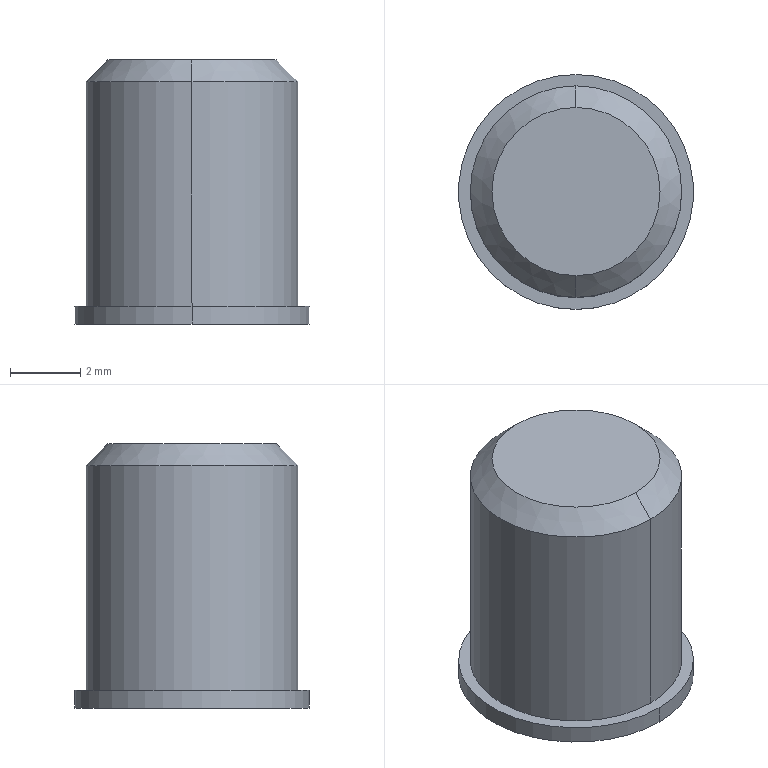Component | SolidWorks | NewCurveBenderHG20Slider-DoubleWheel-1_NewTypeCurveBenderDoubleWheel-1 | 1 solid | 16 faces | box 6.67 x 6.67 x 7.5 mm | volume 204 mm3 | plane 10 | cylinder 4 | cone 2 | commonest cylinder face diameters 6 x2 6.667 x2
STEP:
#1=COLOUR_RGB('',0.7922,0.8196,0.9333);
#2=FILL_AREA_STYLE_COLOUR('',#1);
#3=FILL_AREA_STYLE('',(#2));
#4=SURFACE_STYLE_FILL_AREA(#3);
#5=SURFACE_SIDE_STYLE('',(#4));
#6=SURFACE_STYLE_USAGE(.BOTH.,#5);
#7=PRESENTATION_STYLE_ASSIGNMENT((#6));
#8=CARTESIAN_POINT('',(3.15,1.417,2.082));
#9=VERTEX_POINT('',#8);
#10=CARTESIAN_POINT('',(3.15,1.654,2.082));
#11=VERTEX_POINT('',#10);
#12=CARTESIAN_POINT('',(3.15,1.535,2.082));
#13=DIRECTION('',(-0.,0.,1.));
#14=DIRECTION('',(0.,-1.,0.));
#15=AXIS2_PLACEMENT_3D('',#12,#13,#14);
#16=CIRCLE('',#15,0.1181);
#17=EDGE_CURVE('',#9,#11,#16,.T.);
#18=ORIENTED_EDGE('',*,*,#17,.T.);
#19=CARTESIAN_POINT('',(3.15,1.654,2.333));
#20=VERTEX_POINT('',#19);
#21=CARTESIAN_POINT('',(3.15,1.654,2.062));
#22=DIRECTION('',(-0.,0.,1.));
#23=VECTOR('',#22,39.37);
#24=LINE('',#21,#23);
#25=EDGE_CURVE('',#11,#20,#24,.T.);
#26=ORIENTED_EDGE('',*,*,#25,.T.);
#27=CARTESIAN_POINT('',(3.15,1.417,2.333));
#28=VERTEX_POINT('',#27);
#29=CARTESIAN_POINT('',(3.15,1.535,2.333));
#30=DIRECTION('',(0.,0.,-1.));
#31=DIRECTION('',(0.,-1.,0.));
#32=AXIS2_PLACEMENT_3D('',#29,#30,#31);
#33=CIRCLE('',#32,0.1181);
#34=EDGE_CURVE('',#20,#28,#33,.T.);
#35=ORIENTED_EDGE('',*,*,#34,.T.);
#36=CARTESIAN_POINT('',(3.15,1.417,2.062));
#37=DIRECTION('',(-0.,0.,1.));
#38=VECTOR('',#37,39.37);
#39=LINE('',#36,#38);
#40=EDGE_CURVE('',#9,#28,#39,.T.);
#41=ORIENTED_EDGE('',*,*,#40,.F.);
#42=EDGE_LOOP('',(#18,#26,#35,#41));
#43=FACE_OUTER_BOUND('',#42,.T.);
#44=CARTESIAN_POINT('',(3.15,1.535,2.062));
#45=DIRECTION('',(-0.,0.,1.));
#46=DIRECTION('',(0.,-1.,0.));
#47=AXIS2_PLACEMENT_3D('',#44,#45,#46);
#48=CYLINDRICAL_SURFACE('',#47,0.1181);
#49=ADVANCED_FACE('',(#43),#48,.T.);
#50=CARTESIAN_POINT('',(3.15,1.629,2.357));
#51=VERTEX_POINT('',#50);
#52=CARTESIAN_POINT('',(3.15,1.441,2.357));
#53=VERTEX_POINT('',#52);
#54=CARTESIAN_POINT('',(3.15,1.535,2.357));
#55=DIRECTION('',(0.,0.,-1.));
#56=DIRECTION('',(0.,1.,0.));
#57=AXIS2_PLACEMENT_3D('',#54,#55,#56);
#58=CIRCLE('',#57,0.09396);
#59=EDGE_CURVE('',#51,#53,#58,.T.);
#60=ORIENTED_EDGE('',*,*,#59,.T.);
#61=CARTESIAN_POINT('',(3.15,1.417,2.333));
#62=DIRECTION('',(0.,-0.7071,-0.7071));
#63=VECTOR('',#62,39.37);
#64=LINE('',#61,#63);
#65=EDGE_CURVE('',#53,#28,#64,.T.);
#66=ORIENTED_EDGE('',*,*,#65,.T.);
#67=ORIENTED_EDGE('',*,*,#34,.F.);
#68=CARTESIAN_POINT('',(3.15,1.654,2.333));
#69=DIRECTION('',(0.,0.7071,-0.7071));
#70=VECTOR('',#69,39.37);
#71=LINE('',#68,#70);
#72=EDGE_CURVE('',#51,#20,#71,.T.);
#73=ORIENTED_EDGE('',*,*,#72,.F.);
#74=EDGE_LOOP('',(#60,#66,#67,#73));
#75=FACE_OUTER_BOUND('',#74,.T.);
#76=CARTESIAN_POINT('',(3.15,1.535,2.333));
#77=DIRECTION('',(0.,0.,-1.));
#78=DIRECTION('',(0.,1.,0.));
#79=AXIS2_PLACEMENT_3D('',#76,#77,#78);
#80=CONICAL_SURFACE('',#79,0.1181,0.7854);
#81=ADVANCED_FACE('',(#75),#80,.T.);
#82=CARTESIAN_POINT('',(3.15,1.404,2.062));
#83=VERTEX_POINT('',#82);
#84=CARTESIAN_POINT('',(3.15,1.667,2.062));
#85=VERTEX_POINT('',#84);
#86=CARTESIAN_POINT('',(3.15,1.535,2.062));
#87=DIRECTION('',(-0.,0.,1.));
#88=DIRECTION('',(0.,-1.,0.));
#89=AXIS2_PLACEMENT_3D('',#86,#87,#88);
#90=CIRCLE('',#89,0.1312);
#91=EDGE_CURVE('',#83,#85,#90,.T.);
#92=ORIENTED_EDGE('',*,*,#91,.T.);
#93=CARTESIAN_POINT('',(3.15,1.667,2.082));
#94=VERTEX_POINT('',#93);
#95=CARTESIAN_POINT('',(3.15,1.667,2.062));
#96=DIRECTION('',(-0.,0.,1.));
#97=VECTOR('',#96,39.37);
#98=LINE('',#95,#97);
#99=EDGE_CURVE('',#85,#94,#98,.T.);
#100=ORIENTED_EDGE('',*,*,#99,.T.);
#101=CARTESIAN_POINT('',(3.15,1.404,2.082));
#102=VERTEX_POINT('',#101);
#103=CARTESIAN_POINT('',(3.15,1.535,2.082));
#104=DIRECTION('',(0.,0.,-1.));
#105=DIRECTION('',(0.,-1.,0.));
#106=AXIS2_PLACEMENT_3D('',#103,#104,#105);
#107=CIRCLE('',#106,0.1312);
#108=EDGE_CURVE('',#94,#102,#107,.T.);
#109=ORIENTED_EDGE('',*,*,#108,.T.);
#110=CARTESIAN_POINT('',(3.15,1.404,2.062));
#111=DIRECTION('',(-0.,0.,1.));
#112=VECTOR('',#111,39.37);
#113=LINE('',#110,#112);
#114=EDGE_CURVE('',#83,#102,#113,.T.);
#115=ORIENTED_EDGE('',*,*,#114,.F.);
#116=EDGE_LOOP('',(#92,#100,#109,#115));
#117=FACE_OUTER_BOUND('',#116,.T.);
#118=CARTESIAN_POINT('',(3.15,1.535,2.062));
#119=DIRECTION('',(-0.,0.,1.));
#120=DIRECTION('',(0.,-1.,0.));
#121=AXIS2_PLACEMENT_3D('',#118,#119,#120);
#122=CYLINDRICAL_SURFACE('',#121,0.1312);
#123=ADVANCED_FACE('',(#117),#122,.T.);
#124=ORIENTED_EDGE('',*,*,#25,.F.);
#125=CARTESIAN_POINT('',(3.15,1.535,2.082));
#126=DIRECTION('',(-0.,0.,1.));
#127=DIRECTION('',(0.,-1.,0.));
#128=AXIS2_PLACEMENT_3D('',#125,#126,#127);
#129=CIRCLE('',#128,0.1181);
#130=EDGE_CURVE('',#11,#9,#129,.T.);
#131=ORIENTED_EDGE('',*,*,#130,.T.);
#132=ORIENTED_EDGE('',*,*,#40,.T.);
#133=CARTESIAN_POINT('',(3.15,1.535,2.333));
#134=DIRECTION('',(0.,0.,-1.));
#135=DIRECTION('',(0.,-1.,0.));
#136=AXIS2_PLACEMENT_3D('',#133,#134,#135);
#137=CIRCLE('',#136,0.1181);
#138=EDGE_CURVE('',#28,#20,#137,.T.);
#139=ORIENTED_EDGE('',*,*,#138,.T.);
#140=EDGE_LOOP('',(#124,#131,#132,#139));
#141=FACE_OUTER_BOUND('',#140,.T.);
#142=CARTESIAN_POINT('',(3.15,1.535,2.062));
#143=DIRECTION('',(-0.,0.,1.));
#144=DIRECTION('',(0.,-1.,0.));
#145=AXIS2_PLACEMENT_3D('',#142,#143,#144);
#146=CYLINDRICAL_SURFACE('',#145,0.1181);
#147=ADVANCED_FACE('',(#141),#146,.T.);
#148=ORIENTED_EDGE('',*,*,#65,.F.);
#149=CARTESIAN_POINT('',(3.15,1.535,2.357));
#150=DIRECTION('',(0.,0.,-1.));
#151=DIRECTION('',(0.,1.,0.));
#152=AXIS2_PLACEMENT_3D('',#149,#150,#151);
#153=CIRCLE('',#152,0.09396);
#154=EDGE_CURVE('',#53,#51,#153,.T.);
#155=ORIENTED_EDGE('',*,*,#154,.T.);
#156=ORIENTED_EDGE('',*,*,#72,.T.);
#157=ORIENTED_EDGE('',*,*,#138,.F.);
#158=EDGE_LOOP('',(#148,#155,#156,#157));
#159=FACE_OUTER_BOUND('',#158,.T.);
#160=CARTESIAN_POINT('',(3.15,1.535,2.333));
#161=DIRECTION('',(0.,0.,-1.));
#162=DIRECTION('',(0.,1.,0.));
#163=AXIS2_PLACEMENT_3D('',#160,#161,#162);
#164=CONICAL_SURFACE('',#163,0.1181,0.7854);
#165=ADVANCED_FACE('',(#159),#164,.T.);
#166=ORIENTED_EDGE('',*,*,#17,.F.);
#167=ORIENTED_EDGE('',*,*,#130,.F.);
#168=EDGE_LOOP('',(#166,#167));
#169=FACE_BOUND('',#168,.T.);
#170=CARTESIAN_POINT('',(3.15,1.535,2.082));
#171=DIRECTION('',(0.,0.,-1.));
#172=DIRECTION('',(0.,-1.,0.));
#173=AXIS2_PLACEMENT_3D('',#170,#171,#172);
#174=CIRCLE('',#173,0.1312);
#175=EDGE_CURVE('',#102,#94,#174,.T.);
#176=ORIENTED_EDGE('',*,*,#175,.F.);
#177=ORIENTED_EDGE('',*,*,#108,.F.);
#178=EDGE_LOOP('',(#176,#177));
#179=FACE_OUTER_BOUND('',#178,.T.);
#180=CARTESIAN_POINT('',(3.031,1.535,2.082));
#181=DIRECTION('',(0.,0.,-1.));
#182=DIRECTION('',(0.,1.,0.));
#183=AXIS2_PLACEMENT_3D('',#180,#181,#182);
#184=PLANE('',#183);
#185=ADVANCED_FACE('',(#169,#179),#184,.F.);
#186=ORIENTED_EDGE('',*,*,#59,.F.);
#187=ORIENTED_EDGE('',*,*,#154,.F.);
#188=EDGE_LOOP('',(#186,#187));
#189=FACE_OUTER_BOUND('',#188,.T.);
#190=CARTESIAN_POINT('',(3.15,1.535,2.357));
#191=DIRECTION('',(0.,0.,-1.));
#192=DIRECTION('',(0.,1.,0.));
#193=AXIS2_PLACEMENT_3D('',#190,#191,#192);
#194=PLANE('',#193);
#195=ADVANCED_FACE('',(#189),#194,.F.);
#196=ORIENTED_EDGE('',*,*,#99,.F.);
#197=CARTESIAN_POINT('',(3.15,1.535,2.062));
#198=DIRECTION('',(-0.,0.,1.));
#199=DIRECTION('',(0.,-1.,0.));
#200=AXIS2_PLACEMENT_3D('',#197,#198,#199);
#201=CIRCLE('',#200,0.1312);
#202=EDGE_CURVE('',#85,#83,#201,.T.);
#203=ORIENTED_EDGE('',*,*,#202,.T.);
#204=ORIENTED_EDGE('',*,*,#114,.T.);
#205=ORIENTED_EDGE('',*,*,#175,.T.);
#206=EDGE_LOOP('',(#196,#203,#204,#205));
#207=FACE_OUTER_BOUND('',#206,.T.);
#208=CARTESIAN_POINT('',(3.15,1.535,2.062));
#209=DIRECTION('',(-0.,0.,1.));
#210=DIRECTION('',(0.,-1.,0.));
#211=AXIS2_PLACEMENT_3D('',#208,#209,#210);
#212=CYLINDRICAL_SURFACE('',#211,0.1312);
#213=ADVANCED_FACE('',(#207),#212,.T.);
#214=ORIENTED_EDGE('',*,*,#91,.F.);
#215=ORIENTED_EDGE('',*,*,#202,.F.);
#216=EDGE_LOOP('',(#214,#215));
#217=FACE_OUTER_BOUND('',#216,.T.);
#218=CARTESIAN_POINT('',(3.15,1.454,2.062));
#219=VERTEX_POINT('',#218);
#220=CARTESIAN_POINT('',(3.079,1.495,2.062));
#221=VERTEX_POINT('',#220);
#222=CARTESIAN_POINT('',(3.15,1.454,2.062));
#223=DIRECTION('',(-0.866,0.5,-0.));
#224=VECTOR('',#223,39.37);
#225=LINE('',#222,#224);
#226=EDGE_CURVE('',#219,#221,#225,.T.);
#227=ORIENTED_EDGE('',*,*,#226,.F.);
#228=CARTESIAN_POINT('',(3.22,1.495,2.062));
#229=VERTEX_POINT('',#228);
#230=CARTESIAN_POINT('',(3.22,1.495,2.062));
#231=DIRECTION('',(-0.866,-0.5,-0.));
#232=VECTOR('',#231,39.37);
#233=LINE('',#230,#232);
#234=EDGE_CURVE('',#229,#219,#233,.T.);
#235=ORIENTED_EDGE('',*,*,#234,.F.);
#236=CARTESIAN_POINT('',(3.22,1.576,2.062));
#237=VERTEX_POINT('',#236);
#238=CARTESIAN_POINT('',(3.22,1.535,2.062));
#239=DIRECTION('',(0.,-1.,0.));
#240=VECTOR('',#239,39.37);
#241=LINE('',#238,#240);
#242=EDGE_CURVE('',#237,#229,#241,.T.);
#243=ORIENTED_EDGE('',*,*,#242,.F.);
#244=CARTESIAN_POINT('',(3.15,1.617,2.062));
#245=VERTEX_POINT('',#244);
#246=CARTESIAN_POINT('',(3.15,1.617,2.062));
#247=DIRECTION('',(0.866,-0.5,0.));
#248=VECTOR('',#247,39.37);
#249=LINE('',#246,#248);
#250=EDGE_CURVE('',#245,#237,#249,.T.);
#251=ORIENTED_EDGE('',*,*,#250,.F.);
#252=CARTESIAN_POINT('',(3.079,1.576,2.062));
#253=VERTEX_POINT('',#252);
#254=CARTESIAN_POINT('',(3.079,1.576,2.062));
#255=DIRECTION('',(0.866,0.5,0.));
#256=VECTOR('',#255,39.37);
#257=LINE('',#254,#256);
#258=EDGE_CURVE('',#253,#245,#257,.T.);
#259=ORIENTED_EDGE('',*,*,#258,.F.);
#260=CARTESIAN_POINT('',(3.079,1.535,2.062));
#261=DIRECTION('',(0.,1.,0.));
#262=VECTOR('',#261,39.37);
#263=LINE('',#260,#262);
#264=EDGE_CURVE('',#221,#253,#263,.T.);
#265=ORIENTED_EDGE('',*,*,#264,.F.);
#266=EDGE_LOOP('',(#227,#235,#243,#251,#259,#265));
#267=FACE_BOUND('',#266,.T.);
#268=CARTESIAN_POINT('',(3.018,1.535,2.062));
#269=DIRECTION('',(-0.,0.,1.));
#270=DIRECTION('',(0.,-1.,0.));
#271=AXIS2_PLACEMENT_3D('',#268,#269,#270);
#272=PLANE('',#271);
#273=ADVANCED_FACE('',(#217,#267),#272,.F.);
#274=ORIENTED_EDGE('',*,*,#264,.T.);
#275=CARTESIAN_POINT('',(3.079,1.576,2.092));
#276=VERTEX_POINT('',#275);
#277=CARTESIAN_POINT('',(3.079,1.576,2.092));
#278=DIRECTION('',(0.,0.,-1.));
#279=VECTOR('',#278,39.37);
#280=LINE('',#277,#279);
#281=EDGE_CURVE('',#276,#253,#280,.T.);
#282=ORIENTED_EDGE('',*,*,#281,.F.);
#283=CARTESIAN_POINT('',(3.079,1.495,2.092));
#284=VERTEX_POINT('',#283);
#285=CARTESIAN_POINT('',(3.079,1.495,2.092));
#286=DIRECTION('',(0.,1.,0.));
#287=VECTOR('',#286,39.37);
#288=LINE('',#285,#287);
#289=EDGE_CURVE('',#284,#276,#288,.T.);
#290=ORIENTED_EDGE('',*,*,#289,.F.);
#291=CARTESIAN_POINT('',(3.079,1.495,2.092));
#292=DIRECTION('',(-0.,0.,1.));
#293=VECTOR('',#292,39.37);
#294=LINE('',#291,#293);
#295=EDGE_CURVE('',#221,#284,#294,.T.);
#296=ORIENTED_EDGE('',*,*,#295,.F.);
#297=EDGE_LOOP('',(#274,#282,#290,#296));
#298=FACE_OUTER_BOUND('',#297,.T.);
#299=CARTESIAN_POINT('',(3.079,1.495,2.092));
#300=DIRECTION('',(-1.,0.,-0.));
#301=DIRECTION('',(0.,1.,0.));
#302=AXIS2_PLACEMENT_3D('',#299,#300,#301);
#303=PLANE('',#302);
#304=ADVANCED_FACE('',(#298),#303,.F.);
#305=ORIENTED_EDGE('',*,*,#295,.T.);
#306=CARTESIAN_POINT('',(3.15,1.454,2.092));
#307=VERTEX_POINT('',#306);
#308=CARTESIAN_POINT('',(3.15,1.454,2.092));
#309=DIRECTION('',(-0.866,0.5,-0.));
#310=VECTOR('',#309,39.37);
#311=LINE('',#308,#310);
#312=EDGE_CURVE('',#307,#284,#311,.T.);
#313=ORIENTED_EDGE('',*,*,#312,.F.);
#314=CARTESIAN_POINT('',(3.15,1.454,2.092));
#315=DIRECTION('',(-0.,0.,1.));
#316=VECTOR('',#315,39.37);
#317=LINE('',#314,#316);
#318=EDGE_CURVE('',#219,#307,#317,.T.);
#319=ORIENTED_EDGE('',*,*,#318,.F.);
#320=ORIENTED_EDGE('',*,*,#226,.T.);
#321=EDGE_LOOP('',(#305,#313,#319,#320));
#322=FACE_OUTER_BOUND('',#321,.T.);
#323=CARTESIAN_POINT('',(3.15,1.454,2.092));
#324=DIRECTION('',(-0.5,-0.866,-0.));
#325=DIRECTION('',(-0.866,0.5,-0.));
#326=AXIS2_PLACEMENT_3D('',#323,#324,#325);
#327=PLANE('',#326);
#328=ADVANCED_FACE('',(#322),#327,.F.);
#329=ORIENTED_EDGE('',*,*,#318,.T.);
#330=CARTESIAN_POINT('',(3.22,1.495,2.092));
#331=VERTEX_POINT('',#330);
#332=CARTESIAN_POINT('',(3.22,1.495,2.092));
#333=DIRECTION('',(-0.866,-0.5,-0.));
#334=VECTOR('',#333,39.37);
#335=LINE('',#332,#334);
#336=EDGE_CURVE('',#331,#307,#335,.T.);
#337=ORIENTED_EDGE('',*,*,#336,.F.);
#338=CARTESIAN_POINT('',(3.22,1.495,2.092));
#339=DIRECTION('',(-0.,0.,1.));
#340=VECTOR('',#339,39.37);
#341=LINE('',#338,#340);
#342=EDGE_CURVE('',#229,#331,#341,.T.);
#343=ORIENTED_EDGE('',*,*,#342,.F.);
#344=ORIENTED_EDGE('',*,*,#234,.T.);
#345=EDGE_LOOP('',(#329,#337,#343,#344));
#346=FACE_OUTER_BOUND('',#345,.T.);
#347=CARTESIAN_POINT('',(3.22,1.495,2.092));
#348=DIRECTION('',(0.5,-0.866,0.));
#349=DIRECTION('',(-0.866,-0.5,-0.));
#350=AXIS2_PLACEMENT_3D('',#347,#348,#349);
#351=PLANE('',#350);
#352=ADVANCED_FACE('',(#346),#351,.F.);
#353=ORIENTED_EDGE('',*,*,#342,.T.);
#354=CARTESIAN_POINT('',(3.22,1.576,2.092));
#355=VERTEX_POINT('',#354);
#356=CARTESIAN_POINT('',(3.22,1.576,2.092));
#357=DIRECTION('',(0.,-1.,0.));
#358=VECTOR('',#357,39.37);
#359=LINE('',#356,#358);
#360=EDGE_CURVE('',#355,#331,#359,.T.);
#361=ORIENTED_EDGE('',*,*,#360,.F.);
#362=CARTESIAN_POINT('',(3.22,1.576,2.092));
#363=DIRECTION('',(-0.,0.,1.));
#364=VECTOR('',#363,39.37);
#365=LINE('',#362,#364);
#366=EDGE_CURVE('',#237,#355,#365,.T.);
#367=ORIENTED_EDGE('',*,*,#366,.F.);
#368=ORIENTED_EDGE('',*,*,#242,.T.);
#369=EDGE_LOOP('',(#353,#361,#367,#368));
#370=FACE_OUTER_BOUND('',#369,.T.);
#371=CARTESIAN_POINT('',(3.22,1.576,2.092));
#372=DIRECTION('',(1.,0.,0.));
#373=DIRECTION('',(0.,-1.,0.));
#374=AXIS2_PLACEMENT_3D('',#371,#372,#373);
#375=PLANE('',#374);
#376=ADVANCED_FACE('',(#370),#375,.F.);
#377=ORIENTED_EDGE('',*,*,#366,.T.);
#378=CARTESIAN_POINT('',(3.15,1.617,2.092));
#379=VERTEX_POINT('',#378);
#380=CARTESIAN_POINT('',(3.15,1.617,2.092));
#381=DIRECTION('',(0.866,-0.5,0.));
#382=VECTOR('',#381,39.37);
#383=LINE('',#380,#382);
#384=EDGE_CURVE('',#379,#355,#383,.T.);
#385=ORIENTED_EDGE('',*,*,#384,.F.);
#386=CARTESIAN_POINT('',(3.15,1.617,2.092));
#387=DIRECTION('',(-0.,0.,1.));
#388=VECTOR('',#387,39.37);
#389=LINE('',#386,#388);
#390=EDGE_CURVE('',#245,#379,#389,.T.);
#391=ORIENTED_EDGE('',*,*,#390,.F.);
#392=ORIENTED_EDGE('',*,*,#250,.T.);
#393=EDGE_LOOP('',(#377,#385,#391,#392));
#394=FACE_OUTER_BOUND('',#393,.T.);
#395=CARTESIAN_POINT('',(3.15,1.617,2.092));
#396=DIRECTION('',(0.5,0.866,0.));
#397=DIRECTION('',(0.866,-0.5,0.));
#398=AXIS2_PLACEMENT_3D('',#395,#396,#397);
#399=PLANE('',#398);
#400=ADVANCED_FACE('',(#394),#399,.F.);
#401=ORIENTED_EDGE('',*,*,#390,.T.);
#402=CARTESIAN_POINT('',(3.079,1.576,2.092));
#403=DIRECTION('',(0.866,0.5,0.));
#404=VECTOR('',#403,39.37);
#405=LINE('',#402,#404);
#406=EDGE_CURVE('',#276,#379,#405,.T.);
#407=ORIENTED_EDGE('',*,*,#406,.F.);
#408=ORIENTED_EDGE('',*,*,#281,.T.);
#409=ORIENTED_EDGE('',*,*,#258,.T.);
#410=EDGE_LOOP('',(#401,#407,#408,#409));
#411=FACE_OUTER_BOUND('',#410,.T.);
#412=CARTESIAN_POINT('',(3.079,1.576,2.092));
#413=DIRECTION('',(-0.5,0.866,-0.));
#414=DIRECTION('',(0.866,0.5,0.));
#415=AXIS2_PLACEMENT_3D('',#412,#413,#414);
#416=PLANE('',#415);
#417=ADVANCED_FACE('',(#411),#416,.F.);
#418=ORIENTED_EDGE('',*,*,#336,.T.);
#419=ORIENTED_EDGE('',*,*,#312,.T.);
#420=ORIENTED_EDGE('',*,*,#289,.T.);
#421=ORIENTED_EDGE('',*,*,#406,.T.);
#422=ORIENTED_EDGE('',*,*,#384,.T.);
#423=ORIENTED_EDGE('',*,*,#360,.T.);
#424=EDGE_LOOP('',(#418,#419,#420,#421,#422,#423));
#425=FACE_OUTER_BOUND('',#424,.T.);
#426=CARTESIAN_POINT('',(3.15,1.535,2.092));
#427=DIRECTION('',(0.,0.,-1.));
#428=DIRECTION('',(0.,1.,0.));
#429=AXIS2_PLACEMENT_3D('',#426,#427,#428);
#430=PLANE('',#429);
#431=ADVANCED_FACE('',(#425),#430,.T.);
#432=CLOSED_SHELL('',(#49,#81,#123,#147,#165,#185,#195,#213,#273,#304,#328,#352,#376,#400,#417,#431));
#433=MANIFOLD_SOLID_BREP('',#432);
#434=STYLED_ITEM('',(#7),#433);
#435=PRESENTATION_LAYER_ASSIGNMENT('','',(#434));
#436=(LENGTH_UNIT()NAMED_UNIT(*)SI_UNIT($,.METRE.));
#437=LENGTH_MEASURE_WITH_UNIT(LENGTH_MEASURE(0.0254),#436);
#438=DIMENSIONAL_EXPONENTS(1.,0.,0.,0.,0.,0.,0.);
#439=(CONVERSION_BASED_UNIT('',#437)LENGTH_UNIT()NAMED_UNIT(#438));
#440=UNCERTAINTY_MEASURE_WITH_UNIT(LENGTH_MEASURE(0.00001),#439,'','');
#441=(NAMED_UNIT(*)PLANE_ANGLE_UNIT()SI_UNIT($,.RADIAN.));
#442=(NAMED_UNIT(*)SI_UNIT($,.STERADIAN.)SOLID_ANGLE_UNIT());
#443=(GEOMETRIC_REPRESENTATION_CONTEXT(3)GLOBAL_UNCERTAINTY_ASSIGNED_CONTEXT((#440))GLOBAL_UNIT_ASSIGNED_CONTEXT((#439,#441,#442))REPRESENTATION_CONTEXT('',''));
#444=MECHANICAL_DESIGN_GEOMETRIC_PRESENTATION_REPRESENTATION('',(#434),#443);
#445=CARTESIAN_POINT('',(0.,0.,0.));
#446=DIRECTION('',(0.,0.,1.));
#447=DIRECTION('',(1.,0.,0.));
#448=AXIS2_PLACEMENT_3D('',#445,#446,#447);
#449=(LENGTH_UNIT()NAMED_UNIT(*)SI_UNIT($,.METRE.));
#450=LENGTH_MEASURE_WITH_UNIT(LENGTH_MEASURE(0.0254),#449);
#451=DIMENSIONAL_EXPONENTS(1.,0.,0.,0.,0.,0.,0.);
#452=(CONVERSION_BASED_UNIT('',#450)LENGTH_UNIT()NAMED_UNIT(#451));
#453=UNCERTAINTY_MEASURE_WITH_UNIT(LENGTH_MEASURE(0.00001),#452,'','');
#454=(NAMED_UNIT(*)PLANE_ANGLE_UNIT()SI_UNIT($,.RADIAN.));
#455=(NAMED_UNIT(*)SI_UNIT($,.STERADIAN.)SOLID_ANGLE_UNIT());
#456=(GEOMETRIC_REPRESENTATION_CONTEXT(3)GLOBAL_UNCERTAINTY_ASSIGNED_CONTEXT((#453))GLOBAL_UNIT_ASSIGNED_CONTEXT((#452,#454,#455))REPRESENTATION_CONTEXT('',''));
#457=ADVANCED_BREP_SHAPE_REPRESENTATION('',(#433,#448),#456);